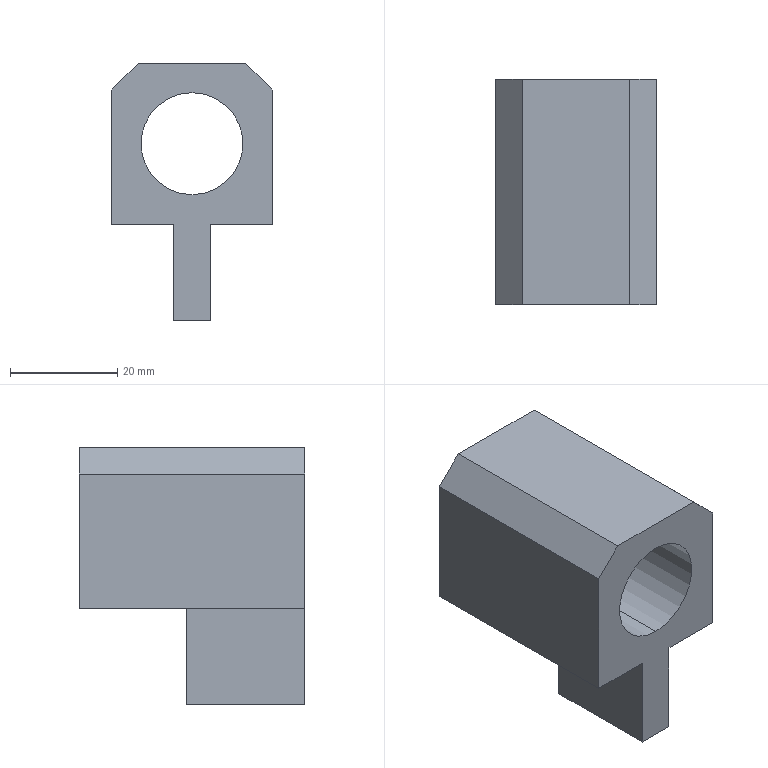Component | SolidWorks | STB-08-021-1 | 1 solid | 22 faces | box 30 x 42 x 48 mm | volume 27411 mm3 | plane 12 | cylinder 6 | cone 4 | commonest cylinder face diameters 3.3 x4 19 x2
build123d program:
from build123d import *

# Parameters (mm, degrees)
SKETCH1_W             = 30
SKETCH1_H             = 48
BOSS_EXTRUDE1_DEPTH   = 21
CUT_EXTRUDE1_REACH    = 52.646
SKETCH2_R             = 9.5
CUT_EXTRUDE2_REACH    = 52.646
SKETCH3_W             = 11.5
SKETCH3_H             = 18
M4_TAPPED_HOLE1_D     = 3.3
M4_TAPPED_HOLE1_DEPTH = 11.5
M4_TAPPED_HOLE1_TIP   = 0.9914
SKETCH7_W             = 7
SKETCH7_H             = 20
CUT_EXTRUDE4_DEPTH    = 18
CHAMFER1_SIZE         = 5


with BuildPart() as part:
    # Sketch1 → Boss-Extrude1 (new, symmetric)
    with BuildSketch(Plane(origin=(0, 0, 0), x_dir=(1, 0, 0), z_dir=(0, 1, 0))):
        Rectangle(SKETCH1_W, SKETCH1_H)
    extrude(amount=BOSS_EXTRUDE1_DEPTH, both=True)

    # Sketch2 → Cut-Extrude1 (cut, up to next)
    with BuildSketch(Plane(origin=(0, 21, 0), x_dir=(1, 0, 0), z_dir=(0, 1, 0)), mode=Mode.PRIVATE) as cut_extrude1_sk1:
        with Locations(Location((0, -9, 0), (0, 0, 270))):
            Circle(SKETCH2_R)
    cut_extrude1_tool1 = extrude(cut_extrude1_sk1.sketch, amount=-CUT_EXTRUDE1_REACH, mode=Mode.PRIVATE) & part.part
    add(cut_extrude1_tool1.solids().sort_by_distance((0, 21, 9))[0], mode=Mode.SUBTRACT)

    # Sketch3 → Cut-Extrude2 (cut, up to next)
    with BuildSketch(Plane(origin=(0, 21, 0), x_dir=(1, 0, 0), z_dir=(0, 1, 0)), mode=Mode.PRIVATE) as cut_extrude2_sk1:
        with Locations((-9.25, 15)):
            Rectangle(SKETCH3_W, SKETCH3_H)
    cut_extrude2_tool1 = extrude(cut_extrude2_sk1.sketch, amount=-CUT_EXTRUDE2_REACH, mode=Mode.PRIVATE) & part.part
    # Sketch3 → Cut-Extrude2 (cut, up to next)
    with BuildSketch(Plane(origin=(0, 21, 0), x_dir=(1, 0, 0), z_dir=(0, 1, 0)), mode=Mode.PRIVATE) as cut_extrude2_sk2:
        with Locations((9.25, 15)):
            Rectangle(SKETCH3_W, SKETCH3_H)
    cut_extrude2_tool2 = extrude(cut_extrude2_sk2.sketch, amount=-CUT_EXTRUDE2_REACH, mode=Mode.PRIVATE) & part.part
    add(cut_extrude2_tool1.solids().sort_by_distance((-9.25, 21, -15))[0], mode=Mode.SUBTRACT)
    add(cut_extrude2_tool2.solids().sort_by_distance((9.25, 21, -15))[0], mode=Mode.SUBTRACT)

    # M4 Tapped Hole1
    with Locations(Plane(origin=(0, 0, -24), x_dir=(-1, 0, 0), z_dir=(0, 0, -1))):
        with Locations((0, -15), (0, -5)):
            Hole(M4_TAPPED_HOLE1_D / 2, depth=M4_TAPPED_HOLE1_DEPTH)
            with Locations((0, 0, -(M4_TAPPED_HOLE1_DEPTH + M4_TAPPED_HOLE1_TIP / 2))):  # 118° drill point
                Cone(0, M4_TAPPED_HOLE1_D / 2, M4_TAPPED_HOLE1_TIP, mode=Mode.SUBTRACT)

    # Sketch7 → Cut-Extrude4 (cut)
    with BuildSketch(Plane(origin=(0, 0, -24), x_dir=(-1, 0, 0), z_dir=(0, 0, -1))):
        with Locations((0, 11)):
            Rectangle(SKETCH7_W, SKETCH7_H)
    extrude(amount=-CUT_EXTRUDE4_DEPTH, mode=Mode.SUBTRACT)

    # Chamfer1
    chamfer1_edges = [part.edges().sort_by_distance(p)[0] for p in [
        (15, 0, 24),
        (-15, 0, 24),
    ]]
    chamfer(chamfer1_edges, length=CHAMFER1_SIZE)


solid = part.part

# Placed as in the assembly
solid = solid.moved(Location((-149.904, 281.499, -21), (0, 0, 0)))
STEP:
#1=COLOUR_RGB('',0.7922,0.8196,0.9333);
#2=FILL_AREA_STYLE_COLOUR('',#1);
#3=FILL_AREA_STYLE('',(#2));
#4=SURFACE_STYLE_FILL_AREA(#3);
#5=SURFACE_SIDE_STYLE('',(#4));
#6=SURFACE_STYLE_USAGE(.BOTH.,#5);
#7=PRESENTATION_STYLE_ASSIGNMENT((#6));
#8=CARTESIAN_POINT('',(-5.837,10.492,-1.319));
#9=VERTEX_POINT('',#8);
#10=CARTESIAN_POINT('',(-5.967,10.492,-1.319));
#11=VERTEX_POINT('',#10);
#12=CARTESIAN_POINT('',(-5.902,10.492,-1.319));
#13=DIRECTION('',(0.,0.,-1.));
#14=DIRECTION('',(-1.,0.,0.));
#15=AXIS2_PLACEMENT_3D('',#12,#13,#14);
#16=CIRCLE('',#15,0.06496);
#17=EDGE_CURVE('',#9,#11,#16,.T.);
#18=ORIENTED_EDGE('',*,*,#17,.F.);
#19=CARTESIAN_POINT('',(-5.837,10.492,-1.772));
#20=VERTEX_POINT('',#19);
#21=CARTESIAN_POINT('',(-5.837,10.492,-1.772));
#22=DIRECTION('',(0.,0.,-1.));
#23=VECTOR('',#22,39.37);
#24=LINE('',#21,#23);
#25=EDGE_CURVE('',#9,#20,#24,.T.);
#26=ORIENTED_EDGE('',*,*,#25,.T.);
#27=CARTESIAN_POINT('',(-5.967,10.492,-1.772));
#28=VERTEX_POINT('',#27);
#29=CARTESIAN_POINT('',(-5.902,10.492,-1.772));
#30=DIRECTION('',(0.,0.,-1.));
#31=DIRECTION('',(-1.,0.,0.));
#32=AXIS2_PLACEMENT_3D('',#29,#30,#31);
#33=CIRCLE('',#32,0.06496);
#34=EDGE_CURVE('',#20,#28,#33,.T.);
#35=ORIENTED_EDGE('',*,*,#34,.T.);
#36=CARTESIAN_POINT('',(-5.967,10.492,-1.772));
#37=DIRECTION('',(0.,0.,-1.));
#38=VECTOR('',#37,39.37);
#39=LINE('',#36,#38);
#40=EDGE_CURVE('',#11,#28,#39,.T.);
#41=ORIENTED_EDGE('',*,*,#40,.F.);
#42=EDGE_LOOP('',(#18,#26,#35,#41));
#43=FACE_OUTER_BOUND('',#42,.T.);
#44=CARTESIAN_POINT('',(-5.902,10.492,-1.772));
#45=DIRECTION('',(0.,0.,-1.));
#46=DIRECTION('',(-1.,0.,0.));
#47=AXIS2_PLACEMENT_3D('',#44,#45,#46);
#48=CYLINDRICAL_SURFACE('',#47,0.06496);
#49=ADVANCED_FACE('',(#43),#48,.F.);
#50=CARTESIAN_POINT('',(-5.902,10.492,-1.28));
#51=VERTEX_POINT('',#50);
#52=CARTESIAN_POINT('',(-5.967,10.492,-1.319));
#53=DIRECTION('',(-0.8572,0.,-0.515));
#54=VECTOR('',#53,39.37);
#55=LINE('',#52,#54);
#56=EDGE_CURVE('',#51,#11,#55,.T.);
#57=ORIENTED_EDGE('',*,*,#56,.F.);
#58=CARTESIAN_POINT('',(-5.837,10.492,-1.319));
#59=DIRECTION('',(0.8572,0.,-0.515));
#60=VECTOR('',#59,39.37);
#61=LINE('',#58,#60);
#62=EDGE_CURVE('',#51,#9,#61,.T.);
#63=ORIENTED_EDGE('',*,*,#62,.T.);
#64=ORIENTED_EDGE('',*,*,#17,.T.);
#65=EDGE_LOOP('',(#57,#63,#64));
#66=FACE_OUTER_BOUND('',#65,.T.);
#67=CARTESIAN_POINT('',(-5.902,10.492,-1.319));
#68=DIRECTION('',(0.,0.,-1.));
#69=DIRECTION('',(-1.,0.,0.));
#70=AXIS2_PLACEMENT_3D('',#67,#68,#69);
#71=CONICAL_SURFACE('',#70,0.06496,1.03);
#72=ADVANCED_FACE('',(#66),#71,.F.);
#73=CARTESIAN_POINT('',(-5.837,10.886,-1.319));
#74=VERTEX_POINT('',#73);
#75=CARTESIAN_POINT('',(-5.967,10.886,-1.319));
#76=VERTEX_POINT('',#75);
#77=CARTESIAN_POINT('',(-5.902,10.886,-1.319));
#78=DIRECTION('',(0.,0.,-1.));
#79=DIRECTION('',(-1.,0.,0.));
#80=AXIS2_PLACEMENT_3D('',#77,#78,#79);
#81=CIRCLE('',#80,0.06496);
#82=EDGE_CURVE('',#74,#76,#81,.T.);
#83=ORIENTED_EDGE('',*,*,#82,.F.);
#84=CARTESIAN_POINT('',(-5.837,10.886,-1.772));
#85=VERTEX_POINT('',#84);
#86=CARTESIAN_POINT('',(-5.837,10.886,-1.772));
#87=DIRECTION('',(0.,0.,-1.));
#88=VECTOR('',#87,39.37);
#89=LINE('',#86,#88);
#90=EDGE_CURVE('',#74,#85,#89,.T.);
#91=ORIENTED_EDGE('',*,*,#90,.T.);
#92=CARTESIAN_POINT('',(-5.967,10.886,-1.772));
#93=VERTEX_POINT('',#92);
#94=CARTESIAN_POINT('',(-5.902,10.886,-1.772));
#95=DIRECTION('',(0.,0.,-1.));
#96=DIRECTION('',(-1.,0.,0.));
#97=AXIS2_PLACEMENT_3D('',#94,#95,#96);
#98=CIRCLE('',#97,0.06496);
#99=EDGE_CURVE('',#85,#93,#98,.T.);
#100=ORIENTED_EDGE('',*,*,#99,.T.);
#101=CARTESIAN_POINT('',(-5.967,10.886,-1.772));
#102=DIRECTION('',(0.,0.,-1.));
#103=VECTOR('',#102,39.37);
#104=LINE('',#101,#103);
#105=EDGE_CURVE('',#76,#93,#104,.T.);
#106=ORIENTED_EDGE('',*,*,#105,.F.);
#107=EDGE_LOOP('',(#83,#91,#100,#106));
#108=FACE_OUTER_BOUND('',#107,.T.);
#109=CARTESIAN_POINT('',(-5.902,10.886,-1.772));
#110=DIRECTION('',(0.,0.,-1.));
#111=DIRECTION('',(-1.,0.,0.));
#112=AXIS2_PLACEMENT_3D('',#109,#110,#111);
#113=CYLINDRICAL_SURFACE('',#112,0.06496);
#114=ADVANCED_FACE('',(#108),#113,.F.);
#115=CARTESIAN_POINT('',(-5.902,10.886,-1.28));
#116=VERTEX_POINT('',#115);
#117=CARTESIAN_POINT('',(-5.967,10.886,-1.319));
#118=DIRECTION('',(-0.8572,0.,-0.515));
#119=VECTOR('',#118,39.37);
#120=LINE('',#117,#119);
#121=EDGE_CURVE('',#116,#76,#120,.T.);
#122=ORIENTED_EDGE('',*,*,#121,.F.);
#123=CARTESIAN_POINT('',(-5.837,10.886,-1.319));
#124=DIRECTION('',(0.8572,0.,-0.515));
#125=VECTOR('',#124,39.37);
#126=LINE('',#123,#125);
#127=EDGE_CURVE('',#116,#74,#126,.T.);
#128=ORIENTED_EDGE('',*,*,#127,.T.);
#129=ORIENTED_EDGE('',*,*,#82,.T.);
#130=EDGE_LOOP('',(#122,#128,#129));
#131=FACE_OUTER_BOUND('',#130,.T.);
#132=CARTESIAN_POINT('',(-5.902,10.886,-1.319));
#133=DIRECTION('',(0.,0.,-1.));
#134=DIRECTION('',(-1.,0.,0.));
#135=AXIS2_PLACEMENT_3D('',#132,#133,#134);
#136=CONICAL_SURFACE('',#135,0.06496,1.03);
#137=ADVANCED_FACE('',(#131),#136,.F.);
#138=CARTESIAN_POINT('',(-5.902,10.256,-0.09843));
#139=VERTEX_POINT('',#138);
#140=CARTESIAN_POINT('',(-5.902,10.256,-0.8465));
#141=VERTEX_POINT('',#140);
#142=CARTESIAN_POINT('',(-5.902,10.256,-0.4724));
#143=DIRECTION('',(0.,-1.,0.));
#144=DIRECTION('',(0.,0.,1.));
#145=AXIS2_PLACEMENT_3D('',#142,#143,#144);
#146=CIRCLE('',#145,0.374);
#147=EDGE_CURVE('',#139,#141,#146,.T.);
#148=ORIENTED_EDGE('',*,*,#147,.T.);
#149=CARTESIAN_POINT('',(-5.902,11.909,-0.8465));
#150=VERTEX_POINT('',#149);
#151=CARTESIAN_POINT('',(-5.902,10.256,-0.8465));
#152=DIRECTION('',(0.,1.,0.));
#153=VECTOR('',#152,39.37);
#154=LINE('',#151,#153);
#155=EDGE_CURVE('',#141,#150,#154,.T.);
#156=ORIENTED_EDGE('',*,*,#155,.T.);
#157=CARTESIAN_POINT('',(-5.902,11.909,-0.09843));
#158=VERTEX_POINT('',#157);
#159=CARTESIAN_POINT('',(-5.902,11.909,-0.4724));
#160=DIRECTION('',(0.,1.,0.));
#161=DIRECTION('',(0.,0.,1.));
#162=AXIS2_PLACEMENT_3D('',#159,#160,#161);
#163=CIRCLE('',#162,0.374);
#164=EDGE_CURVE('',#150,#158,#163,.T.);
#165=ORIENTED_EDGE('',*,*,#164,.T.);
#166=CARTESIAN_POINT('',(-5.902,10.256,-0.09843));
#167=DIRECTION('',(0.,1.,0.));
#168=VECTOR('',#167,39.37);
#169=LINE('',#166,#168);
#170=EDGE_CURVE('',#139,#158,#169,.T.);
#171=ORIENTED_EDGE('',*,*,#170,.F.);
#172=EDGE_LOOP('',(#148,#156,#165,#171));
#173=FACE_OUTER_BOUND('',#172,.T.);
#174=CARTESIAN_POINT('',(-5.902,10.256,-0.4724));
#175=DIRECTION('',(0.,1.,0.));
#176=DIRECTION('',(0.,0.,1.));
#177=AXIS2_PLACEMENT_3D('',#174,#175,#176);
#178=CYLINDRICAL_SURFACE('',#177,0.374);
#179=ADVANCED_FACE('',(#173),#178,.F.);
#180=CARTESIAN_POINT('',(-5.902,11.909,-0.4724));
#181=DIRECTION('',(0.,1.,0.));
#182=DIRECTION('',(0.,0.,1.));
#183=AXIS2_PLACEMENT_3D('',#180,#181,#182);
#184=CIRCLE('',#183,0.374);
#185=EDGE_CURVE('',#158,#150,#184,.T.);
#186=ORIENTED_EDGE('',*,*,#185,.F.);
#187=ORIENTED_EDGE('',*,*,#164,.F.);
#188=EDGE_LOOP('',(#186,#187));
#189=FACE_BOUND('',#188,.T.);
#190=CARTESIAN_POINT('',(-6.492,11.909,-1.063));
#191=VERTEX_POINT('',#190);
#192=CARTESIAN_POINT('',(-6.492,11.909,-0.07874));
#193=VERTEX_POINT('',#192);
#194=CARTESIAN_POINT('',(-6.492,11.909,-1.772));
#195=DIRECTION('',(0.,0.,1.));
#196=VECTOR('',#195,39.37);
#197=LINE('',#194,#196);
#198=EDGE_CURVE('',#191,#193,#197,.T.);
#199=ORIENTED_EDGE('',*,*,#198,.T.);
#200=CARTESIAN_POINT('',(-6.295,11.909,0.1181));
#201=VERTEX_POINT('',#200);
#202=CARTESIAN_POINT('',(-6.394,11.909,0.01969));
#203=DIRECTION('',(0.7071,0.,0.7071));
#204=VECTOR('',#203,39.37);
#205=LINE('',#202,#204);
#206=EDGE_CURVE('',#193,#201,#205,.T.);
#207=ORIENTED_EDGE('',*,*,#206,.T.);
#208=CARTESIAN_POINT('',(-5.508,11.909,0.1181));
#209=VERTEX_POINT('',#208);
#210=CARTESIAN_POINT('',(-6.492,11.909,0.1181));
#211=DIRECTION('',(1.,0.,0.));
#212=VECTOR('',#211,39.37);
#213=LINE('',#210,#212);
#214=EDGE_CURVE('',#201,#209,#213,.T.);
#215=ORIENTED_EDGE('',*,*,#214,.T.);
#216=CARTESIAN_POINT('',(-5.311,11.909,-0.07874));
#217=VERTEX_POINT('',#216);
#218=CARTESIAN_POINT('',(-6.,11.909,0.6102));
#219=DIRECTION('',(0.7071,0.,-0.7071));
#220=VECTOR('',#219,39.37);
#221=LINE('',#218,#220);
#222=EDGE_CURVE('',#209,#217,#221,.T.);
#223=ORIENTED_EDGE('',*,*,#222,.T.);
#224=CARTESIAN_POINT('',(-5.311,11.909,-1.063));
#225=VERTEX_POINT('',#224);
#226=CARTESIAN_POINT('',(-5.311,11.909,-1.772));
#227=DIRECTION('',(0.,0.,-1.));
#228=VECTOR('',#227,39.37);
#229=LINE('',#226,#228);
#230=EDGE_CURVE('',#217,#225,#229,.T.);
#231=ORIENTED_EDGE('',*,*,#230,.T.);
#232=CARTESIAN_POINT('',(-6.492,11.909,-1.063));
#233=DIRECTION('',(1.,0.,0.));
#234=VECTOR('',#233,39.37);
#235=LINE('',#232,#234);
#236=EDGE_CURVE('',#191,#225,#235,.T.);
#237=ORIENTED_EDGE('',*,*,#236,.F.);
#238=EDGE_LOOP('',(#199,#207,#215,#223,#231,#237));
#239=FACE_OUTER_BOUND('',#238,.T.);
#240=CARTESIAN_POINT('',(-6.492,11.909,0.1181));
#241=DIRECTION('',(0.,1.,0.));
#242=DIRECTION('',(0.,0.,1.));
#243=AXIS2_PLACEMENT_3D('',#240,#241,#242);
#244=PLANE('',#243);
#245=ADVANCED_FACE('',(#189,#239),#244,.T.);
#246=CARTESIAN_POINT('',(-6.492,10.256,-1.063));
#247=VERTEX_POINT('',#246);
#248=CARTESIAN_POINT('',(-6.492,10.256,-0.07874));
#249=VERTEX_POINT('',#248);
#250=CARTESIAN_POINT('',(-6.492,10.256,-1.772));
#251=DIRECTION('',(0.,0.,1.));
#252=VECTOR('',#251,39.37);
#253=LINE('',#250,#252);
#254=EDGE_CURVE('',#247,#249,#253,.T.);
#255=ORIENTED_EDGE('',*,*,#254,.T.);
#256=CARTESIAN_POINT('',(-6.492,11.909,-0.07874));
#257=DIRECTION('',(0.,1.,0.));
#258=VECTOR('',#257,39.37);
#259=LINE('',#256,#258);
#260=EDGE_CURVE('',#249,#193,#259,.T.);
#261=ORIENTED_EDGE('',*,*,#260,.T.);
#262=ORIENTED_EDGE('',*,*,#198,.F.);
#263=CARTESIAN_POINT('',(-6.492,10.256,-1.063));
#264=DIRECTION('',(0.,1.,0.));
#265=VECTOR('',#264,39.37);
#266=LINE('',#263,#265);
#267=EDGE_CURVE('',#247,#191,#266,.T.);
#268=ORIENTED_EDGE('',*,*,#267,.F.);
#269=EDGE_LOOP('',(#255,#261,#262,#268));
#270=FACE_OUTER_BOUND('',#269,.T.);
#271=CARTESIAN_POINT('',(-6.492,11.909,-1.772));
#272=DIRECTION('',(1.,0.,0.));
#273=DIRECTION('',(0.,0.,-1.));
#274=AXIS2_PLACEMENT_3D('',#271,#272,#273);
#275=PLANE('',#274);
#276=ADVANCED_FACE('',(#270),#275,.F.);
#277=ORIENTED_EDGE('',*,*,#214,.F.);
#278=CARTESIAN_POINT('',(-6.295,10.256,0.1181));
#279=VERTEX_POINT('',#278);
#280=CARTESIAN_POINT('',(-6.295,11.909,0.1181));
#281=DIRECTION('',(0.,-1.,0.));
#282=VECTOR('',#281,39.37);
#283=LINE('',#280,#282);
#284=EDGE_CURVE('',#201,#279,#283,.T.);
#285=ORIENTED_EDGE('',*,*,#284,.T.);
#286=CARTESIAN_POINT('',(-5.508,10.256,0.1181));
#287=VERTEX_POINT('',#286);
#288=CARTESIAN_POINT('',(-6.492,10.256,0.1181));
#289=DIRECTION('',(1.,0.,0.));
#290=VECTOR('',#289,39.37);
#291=LINE('',#288,#290);
#292=EDGE_CURVE('',#279,#287,#291,.T.);
#293=ORIENTED_EDGE('',*,*,#292,.T.);
#294=CARTESIAN_POINT('',(-5.508,11.909,0.1181));
#295=DIRECTION('',(0.,1.,0.));
#296=VECTOR('',#295,39.37);
#297=LINE('',#294,#296);
#298=EDGE_CURVE('',#287,#209,#297,.T.);
#299=ORIENTED_EDGE('',*,*,#298,.T.);
#300=EDGE_LOOP('',(#277,#285,#293,#299));
#301=FACE_OUTER_BOUND('',#300,.T.);
#302=CARTESIAN_POINT('',(-6.492,11.909,0.1181));
#303=DIRECTION('',(0.,0.,-1.));
#304=DIRECTION('',(-1.,0.,0.));
#305=AXIS2_PLACEMENT_3D('',#302,#303,#304);
#306=PLANE('',#305);
#307=ADVANCED_FACE('',(#301),#306,.F.);
#308=ORIENTED_EDGE('',*,*,#230,.F.);
#309=CARTESIAN_POINT('',(-5.311,10.256,-0.07874));
#310=VERTEX_POINT('',#309);
#311=CARTESIAN_POINT('',(-5.311,11.909,-0.07874));
#312=DIRECTION('',(0.,-1.,0.));
#313=VECTOR('',#312,39.37);
#314=LINE('',#311,#313);
#315=EDGE_CURVE('',#217,#310,#314,.T.);
#316=ORIENTED_EDGE('',*,*,#315,.T.);
#317=CARTESIAN_POINT('',(-5.311,10.256,-1.063));
#318=VERTEX_POINT('',#317);
#319=CARTESIAN_POINT('',(-5.311,10.256,-1.772));
#320=DIRECTION('',(0.,0.,-1.));
#321=VECTOR('',#320,39.37);
#322=LINE('',#319,#321);
#323=EDGE_CURVE('',#310,#318,#322,.T.);
#324=ORIENTED_EDGE('',*,*,#323,.T.);
#325=CARTESIAN_POINT('',(-5.311,10.256,-1.063));
#326=DIRECTION('',(0.,1.,0.));
#327=VECTOR('',#326,39.37);
#328=LINE('',#325,#327);
#329=EDGE_CURVE('',#318,#225,#328,.T.);
#330=ORIENTED_EDGE('',*,*,#329,.T.);
#331=EDGE_LOOP('',(#308,#316,#324,#330));
#332=FACE_OUTER_BOUND('',#331,.T.);
#333=CARTESIAN_POINT('',(-5.311,11.909,-1.772));
#334=DIRECTION('',(-1.,0.,0.));
#335=DIRECTION('',(0.,0.,1.));
#336=AXIS2_PLACEMENT_3D('',#333,#334,#335);
#337=PLANE('',#336);
#338=ADVANCED_FACE('',(#332),#337,.F.);
#339=CARTESIAN_POINT('',(-5.902,10.492,-1.772));
#340=DIRECTION('',(0.,0.,-1.));
#341=DIRECTION('',(-1.,0.,0.));
#342=AXIS2_PLACEMENT_3D('',#339,#340,#341);
#343=CIRCLE('',#342,0.06496);
#344=EDGE_CURVE('',#28,#20,#343,.T.);
#345=ORIENTED_EDGE('',*,*,#344,.F.);
#346=ORIENTED_EDGE('',*,*,#34,.F.);
#347=EDGE_LOOP('',(#345,#346));
#348=FACE_BOUND('',#347,.T.);
#349=CARTESIAN_POINT('',(-5.902,10.886,-1.772));
#350=DIRECTION('',(0.,0.,-1.));
#351=DIRECTION('',(-1.,0.,0.));
#352=AXIS2_PLACEMENT_3D('',#349,#350,#351);
#353=CIRCLE('',#352,0.06496);
#354=EDGE_CURVE('',#93,#85,#353,.T.);
#355=ORIENTED_EDGE('',*,*,#354,.F.);
#356=ORIENTED_EDGE('',*,*,#99,.F.);
#357=EDGE_LOOP('',(#355,#356));
#358=FACE_BOUND('',#357,.T.);
#359=CARTESIAN_POINT('',(-6.04,10.256,-1.772));
#360=VERTEX_POINT('',#359);
#361=CARTESIAN_POINT('',(-6.04,11.122,-1.772));
#362=VERTEX_POINT('',#361);
#363=CARTESIAN_POINT('',(-6.04,10.256,-1.772));
#364=DIRECTION('',(0.,1.,0.));
#365=VECTOR('',#364,39.37);
#366=LINE('',#363,#365);
#367=EDGE_CURVE('',#360,#362,#366,.T.);
#368=ORIENTED_EDGE('',*,*,#367,.T.);
#369=CARTESIAN_POINT('',(-5.764,11.122,-1.772));
#370=VERTEX_POINT('',#369);
#371=CARTESIAN_POINT('',(-5.764,11.122,-1.772));
#372=DIRECTION('',(-1.,0.,0.));
#373=VECTOR('',#372,39.37);
#374=LINE('',#371,#373);
#375=EDGE_CURVE('',#370,#362,#374,.T.);
#376=ORIENTED_EDGE('',*,*,#375,.F.);
#377=CARTESIAN_POINT('',(-5.764,10.256,-1.772));
#378=VERTEX_POINT('',#377);
#379=CARTESIAN_POINT('',(-5.764,10.256,-1.772));
#380=DIRECTION('',(0.,1.,0.));
#381=VECTOR('',#380,39.37);
#382=LINE('',#379,#381);
#383=EDGE_CURVE('',#378,#370,#382,.T.);
#384=ORIENTED_EDGE('',*,*,#383,.F.);
#385=CARTESIAN_POINT('',(-6.492,10.256,-1.772));
#386=DIRECTION('',(-1.,0.,0.));
#387=VECTOR('',#386,39.37);
#388=LINE('',#385,#387);
#389=EDGE_CURVE('',#378,#360,#388,.T.);
#390=ORIENTED_EDGE('',*,*,#389,.T.);
#391=EDGE_LOOP('',(#368,#376,#384,#390));
#392=FACE_OUTER_BOUND('',#391,.T.);
#393=CARTESIAN_POINT('',(-6.492,11.909,-1.772));
#394=DIRECTION('',(0.,0.,1.));
#395=DIRECTION('',(1.,0.,0.));
#396=AXIS2_PLACEMENT_3D('',#393,#394,#395);
#397=PLANE('',#396);
#398=ADVANCED_FACE('',(#348,#358,#392),#397,.F.);
#399=ORIENTED_EDGE('',*,*,#147,.F.);
#400=CARTESIAN_POINT('',(-5.902,10.256,-0.4724));
#401=DIRECTION('',(0.,-1.,0.));
#402=DIRECTION('',(0.,0.,1.));
#403=AXIS2_PLACEMENT_3D('',#400,#401,#402);
#404=CIRCLE('',#403,0.374);
#405=EDGE_CURVE('',#141,#139,#404,.T.);
#406=ORIENTED_EDGE('',*,*,#405,.F.);
#407=EDGE_LOOP('',(#399,#406));
#408=FACE_BOUND('',#407,.T.);
#409=ORIENTED_EDGE('',*,*,#292,.F.);
#410=CARTESIAN_POINT('',(-6.295,10.256,0.1181));
#411=DIRECTION('',(-0.7071,0.,-0.7071));
#412=VECTOR('',#411,39.37);
#413=LINE('',#410,#412);
#414=EDGE_CURVE('',#279,#249,#413,.T.);
#415=ORIENTED_EDGE('',*,*,#414,.T.);
#416=ORIENTED_EDGE('',*,*,#254,.F.);
#417=CARTESIAN_POINT('',(-6.04,10.256,-1.063));
#418=VERTEX_POINT('',#417);
#419=CARTESIAN_POINT('',(-6.492,10.256,-1.063));
#420=DIRECTION('',(-1.,0.,-0.));
#421=VECTOR('',#420,39.37);
#422=LINE('',#419,#421);
#423=EDGE_CURVE('',#418,#247,#422,.T.);
#424=ORIENTED_EDGE('',*,*,#423,.F.);
#425=CARTESIAN_POINT('',(-6.04,10.256,-1.772));
#426=DIRECTION('',(-0.,0.,1.));
#427=VECTOR('',#426,39.37);
#428=LINE('',#425,#427);
#429=EDGE_CURVE('',#360,#418,#428,.T.);
#430=ORIENTED_EDGE('',*,*,#429,.F.);
#431=ORIENTED_EDGE('',*,*,#389,.F.);
#432=CARTESIAN_POINT('',(-5.764,10.256,-1.063));
#433=VERTEX_POINT('',#432);
#434=CARTESIAN_POINT('',(-5.764,10.256,-1.772));
#435=DIRECTION('',(-0.,0.,-1.));
#436=VECTOR('',#435,39.37);
#437=LINE('',#434,#436);
#438=EDGE_CURVE('',#433,#378,#437,.T.);
#439=ORIENTED_EDGE('',*,*,#438,.F.);
#440=CARTESIAN_POINT('',(-5.311,10.256,-1.063));
#441=DIRECTION('',(-1.,0.,0.));
#442=VECTOR('',#441,39.37);
#443=LINE('',#440,#442);
#444=EDGE_CURVE('',#318,#433,#443,.T.);
#445=ORIENTED_EDGE('',*,*,#444,.F.);
#446=ORIENTED_EDGE('',*,*,#323,.F.);
#447=CARTESIAN_POINT('',(-5.311,10.256,-0.07874));
#448=DIRECTION('',(-0.7071,0.,0.7071));
#449=VECTOR('',#448,39.37);
#450=LINE('',#447,#449);
#451=EDGE_CURVE('',#310,#287,#450,.T.);
#452=ORIENTED_EDGE('',*,*,#451,.T.);
#453=EDGE_LOOP('',(#409,#415,#416,#424,#430,#431,#439,#445,#446,#452));
#454=FACE_OUTER_BOUND('',#453,.T.);
#455=CARTESIAN_POINT('',(-6.492,10.256,0.1181));
#456=DIRECTION('',(0.,1.,0.));
#457=DIRECTION('',(0.,0.,1.));
#458=AXIS2_PLACEMENT_3D('',#455,#456,#457);
#459=PLANE('',#458);
#460=ADVANCED_FACE('',(#408,#454),#459,.F.);
#461=ORIENTED_EDGE('',*,*,#155,.F.);
#462=ORIENTED_EDGE('',*,*,#405,.T.);
#463=ORIENTED_EDGE('',*,*,#170,.T.);
#464=ORIENTED_EDGE('',*,*,#185,.T.);
#465=EDGE_LOOP('',(#461,#462,#463,#464));
#466=FACE_OUTER_BOUND('',#465,.T.);
#467=CARTESIAN_POINT('',(-5.902,10.256,-0.4724));
#468=DIRECTION('',(0.,1.,0.));
#469=DIRECTION('',(0.,0.,1.));
#470=AXIS2_PLACEMENT_3D('',#467,#468,#469);
#471=CYLINDRICAL_SURFACE('',#470,0.374);
#472=ADVANCED_FACE('',(#466),#471,.F.);
#473=CARTESIAN_POINT('',(-6.04,11.122,-1.063));
#474=VERTEX_POINT('',#473);
#475=CARTESIAN_POINT('',(-6.04,10.256,-1.063));
#476=DIRECTION('',(0.,1.,0.));
#477=VECTOR('',#476,39.37);
#478=LINE('',#475,#477);
#479=EDGE_CURVE('',#418,#474,#478,.T.);
#480=ORIENTED_EDGE('',*,*,#479,.T.);
#481=CARTESIAN_POINT('',(-6.04,11.122,-1.063));
#482=DIRECTION('',(0.,0.,-1.));
#483=VECTOR('',#482,39.37);
#484=LINE('',#481,#483);
#485=EDGE_CURVE('',#474,#362,#484,.T.);
#486=ORIENTED_EDGE('',*,*,#485,.T.);
#487=ORIENTED_EDGE('',*,*,#367,.F.);
#488=ORIENTED_EDGE('',*,*,#429,.T.);
#489=EDGE_LOOP('',(#480,#486,#487,#488));
#490=FACE_OUTER_BOUND('',#489,.T.);
#491=CARTESIAN_POINT('',(-6.04,10.256,-1.772));
#492=DIRECTION('',(1.,0.,0.));
#493=DIRECTION('',(0.,0.,-1.));
#494=AXIS2_PLACEMENT_3D('',#491,#492,#493);
#495=PLANE('',#494);
#496=ADVANCED_FACE('',(#490),#495,.F.);
#497=ORIENTED_EDGE('',*,*,#423,.T.);
#498=ORIENTED_EDGE('',*,*,#267,.T.);
#499=ORIENTED_EDGE('',*,*,#236,.T.);
#500=ORIENTED_EDGE('',*,*,#329,.F.);
#501=ORIENTED_EDGE('',*,*,#444,.T.);
#502=CARTESIAN_POINT('',(-5.764,11.122,-1.063));
#503=VERTEX_POINT('',#502);
#504=CARTESIAN_POINT('',(-5.764,10.256,-1.063));
#505=DIRECTION('',(0.,1.,0.));
#506=VECTOR('',#505,39.37);
#507=LINE('',#504,#506);
#508=EDGE_CURVE('',#433,#503,#507,.T.);
#509=ORIENTED_EDGE('',*,*,#508,.T.);
#510=CARTESIAN_POINT('',(-5.764,11.122,-1.063));
#511=DIRECTION('',(-1.,0.,0.));
#512=VECTOR('',#511,39.37);
#513=LINE('',#510,#512);
#514=EDGE_CURVE('',#503,#474,#513,.T.);
#515=ORIENTED_EDGE('',*,*,#514,.T.);
#516=ORIENTED_EDGE('',*,*,#479,.F.);
#517=EDGE_LOOP('',(#497,#498,#499,#500,#501,#509,#515,#516));
#518=FACE_OUTER_BOUND('',#517,.T.);
#519=CARTESIAN_POINT('',(-6.492,10.256,-1.063));
#520=DIRECTION('',(-0.,0.,1.));
#521=DIRECTION('',(1.,0.,0.));
#522=AXIS2_PLACEMENT_3D('',#519,#520,#521);
#523=PLANE('',#522);
#524=ADVANCED_FACE('',(#518),#523,.F.);
#525=ORIENTED_EDGE('',*,*,#383,.T.);
#526=CARTESIAN_POINT('',(-5.764,11.122,-1.063));
#527=DIRECTION('',(0.,0.,-1.));
#528=VECTOR('',#527,39.37);
#529=LINE('',#526,#528);
#530=EDGE_CURVE('',#503,#370,#529,.T.);
#531=ORIENTED_EDGE('',*,*,#530,.F.);
#532=ORIENTED_EDGE('',*,*,#508,.F.);
#533=ORIENTED_EDGE('',*,*,#438,.T.);
#534=EDGE_LOOP('',(#525,#531,#532,#533));
#535=FACE_OUTER_BOUND('',#534,.T.);
#536=CARTESIAN_POINT('',(-5.764,10.256,-1.772));
#537=DIRECTION('',(-1.,0.,0.));
#538=DIRECTION('',(0.,0.,1.));
#539=AXIS2_PLACEMENT_3D('',#536,#537,#538);
#540=PLANE('',#539);
#541=ADVANCED_FACE('',(#535),#540,.F.);
#542=ORIENTED_EDGE('',*,*,#127,.F.);
#543=ORIENTED_EDGE('',*,*,#121,.T.);
#544=CARTESIAN_POINT('',(-5.902,10.886,-1.319));
#545=DIRECTION('',(0.,0.,-1.));
#546=DIRECTION('',(-1.,0.,0.));
#547=AXIS2_PLACEMENT_3D('',#544,#545,#546);
#548=CIRCLE('',#547,0.06496);
#549=EDGE_CURVE('',#76,#74,#548,.T.);
#550=ORIENTED_EDGE('',*,*,#549,.T.);
#551=EDGE_LOOP('',(#542,#543,#550));
#552=FACE_OUTER_BOUND('',#551,.T.);
#553=CARTESIAN_POINT('',(-5.902,10.886,-1.319));
#554=DIRECTION('',(0.,0.,-1.));
#555=DIRECTION('',(-1.,0.,0.));
#556=AXIS2_PLACEMENT_3D('',#553,#554,#555);
#557=CONICAL_SURFACE('',#556,0.06496,1.03);
#558=ADVANCED_FACE('',(#552),#557,.F.);
#559=ORIENTED_EDGE('',*,*,#90,.F.);
#560=ORIENTED_EDGE('',*,*,#549,.F.);
#561=ORIENTED_EDGE('',*,*,#105,.T.);
#562=ORIENTED_EDGE('',*,*,#354,.T.);
#563=EDGE_LOOP('',(#559,#560,#561,#562));
#564=FACE_OUTER_BOUND('',#563,.T.);
#565=CARTESIAN_POINT('',(-5.902,10.886,-1.772));
#566=DIRECTION('',(0.,0.,-1.));
#567=DIRECTION('',(-1.,0.,0.));
#568=AXIS2_PLACEMENT_3D('',#565,#566,#567);
#569=CYLINDRICAL_SURFACE('',#568,0.06496);
#570=ADVANCED_FACE('',(#564),#569,.F.);
#571=ORIENTED_EDGE('',*,*,#62,.F.);
#572=ORIENTED_EDGE('',*,*,#56,.T.);
#573=CARTESIAN_POINT('',(-5.902,10.492,-1.319));
#574=DIRECTION('',(0.,0.,-1.));
#575=DIRECTION('',(-1.,0.,0.));
#576=AXIS2_PLACEMENT_3D('',#573,#574,#575);
#577=CIRCLE('',#576,0.06496);
#578=EDGE_CURVE('',#11,#9,#577,.T.);
#579=ORIENTED_EDGE('',*,*,#578,.T.);
#580=EDGE_LOOP('',(#571,#572,#579));
#581=FACE_OUTER_BOUND('',#580,.T.);
#582=CARTESIAN_POINT('',(-5.902,10.492,-1.319));
#583=DIRECTION('',(0.,0.,-1.));
#584=DIRECTION('',(-1.,0.,0.));
#585=AXIS2_PLACEMENT_3D('',#582,#583,#584);
#586=CONICAL_SURFACE('',#585,0.06496,1.03);
#587=ADVANCED_FACE('',(#581),#586,.F.);
#588=ORIENTED_EDGE('',*,*,#25,.F.);
#589=ORIENTED_EDGE('',*,*,#578,.F.);
#590=ORIENTED_EDGE('',*,*,#40,.T.);
#591=ORIENTED_EDGE('',*,*,#344,.T.);
#592=EDGE_LOOP('',(#588,#589,#590,#591));
#593=FACE_OUTER_BOUND('',#592,.T.);
#594=CARTESIAN_POINT('',(-5.902,10.492,-1.772));
#595=DIRECTION('',(0.,0.,-1.));
#596=DIRECTION('',(-1.,0.,0.));
#597=AXIS2_PLACEMENT_3D('',#594,#595,#596);
#598=CYLINDRICAL_SURFACE('',#597,0.06496);
#599=ADVANCED_FACE('',(#593),#598,.F.);
#600=ORIENTED_EDGE('',*,*,#375,.T.);
#601=ORIENTED_EDGE('',*,*,#485,.F.);
#602=ORIENTED_EDGE('',*,*,#514,.F.);
#603=ORIENTED_EDGE('',*,*,#530,.T.);
#604=EDGE_LOOP('',(#600,#601,#602,#603));
#605=FACE_OUTER_BOUND('',#604,.T.);
#606=CARTESIAN_POINT('',(-5.764,11.122,-1.063));
#607=DIRECTION('',(0.,-1.,0.));
#608=DIRECTION('',(0.,0.,-1.));
#609=AXIS2_PLACEMENT_3D('',#606,#607,#608);
#610=PLANE('',#609);
#611=ADVANCED_FACE('',(#605),#610,.F.);
#612=ORIENTED_EDGE('',*,*,#206,.F.);
#613=ORIENTED_EDGE('',*,*,#260,.F.);
#614=ORIENTED_EDGE('',*,*,#414,.F.);
#615=ORIENTED_EDGE('',*,*,#284,.F.);
#616=EDGE_LOOP('',(#612,#613,#614,#615));
#617=FACE_OUTER_BOUND('',#616,.T.);
#618=CARTESIAN_POINT('',(-6.295,11.909,0.1181));
#619=DIRECTION('',(0.7071,0.,-0.7071));
#620=DIRECTION('',(-0.7071,0.,-0.7071));
#621=AXIS2_PLACEMENT_3D('',#618,#619,#620);
#622=PLANE('',#621);
#623=ADVANCED_FACE('',(#617),#622,.F.);
#624=ORIENTED_EDGE('',*,*,#222,.F.);
#625=ORIENTED_EDGE('',*,*,#298,.F.);
#626=ORIENTED_EDGE('',*,*,#451,.F.);
#627=ORIENTED_EDGE('',*,*,#315,.F.);
#628=EDGE_LOOP('',(#624,#625,#626,#627));
#629=FACE_OUTER_BOUND('',#628,.T.);
#630=CARTESIAN_POINT('',(-5.311,11.909,-0.07874));
#631=DIRECTION('',(-0.7071,0.,-0.7071));
#632=DIRECTION('',(-0.7071,0.,0.7071));
#633=AXIS2_PLACEMENT_3D('',#630,#631,#632);
#634=PLANE('',#633);
#635=ADVANCED_FACE('',(#629),#634,.F.);
#636=CLOSED_SHELL('',(#49,#72,#114,#137,#179,#245,#276,#307,#338,#398,#460,#472,#496,#524,#541,#558,#570,#587,#599,#611,#623,#635));
#637=MANIFOLD_SOLID_BREP('',#636);
#638=STYLED_ITEM('',(#7),#637);
#639=PRESENTATION_LAYER_ASSIGNMENT('','',(#638));
#640=(LENGTH_UNIT()NAMED_UNIT(*)SI_UNIT($,.METRE.));
#641=LENGTH_MEASURE_WITH_UNIT(LENGTH_MEASURE(0.0254),#640);
#642=DIMENSIONAL_EXPONENTS(1.,0.,0.,0.,0.,0.,0.);
#643=(CONVERSION_BASED_UNIT('',#641)LENGTH_UNIT()NAMED_UNIT(#642));
#644=UNCERTAINTY_MEASURE_WITH_UNIT(LENGTH_MEASURE(0.00001),#643,'','');
#645=(NAMED_UNIT(*)PLANE_ANGLE_UNIT()SI_UNIT($,.RADIAN.));
#646=(NAMED_UNIT(*)SI_UNIT($,.STERADIAN.)SOLID_ANGLE_UNIT());
#647=(GEOMETRIC_REPRESENTATION_CONTEXT(3)GLOBAL_UNCERTAINTY_ASSIGNED_CONTEXT((#644))GLOBAL_UNIT_ASSIGNED_CONTEXT((#643,#645,#646))REPRESENTATION_CONTEXT('',''));
#648=MECHANICAL_DESIGN_GEOMETRIC_PRESENTATION_REPRESENTATION('',(#638),#647);
#649=CARTESIAN_POINT('',(0.,0.,0.));
#650=DIRECTION('',(0.,0.,1.));
#651=DIRECTION('',(1.,0.,0.));
#652=AXIS2_PLACEMENT_3D('',#649,#650,#651);
#653=(LENGTH_UNIT()NAMED_UNIT(*)SI_UNIT($,.METRE.));
#654=LENGTH_MEASURE_WITH_UNIT(LENGTH_MEASURE(0.0254),#653);
#655=DIMENSIONAL_EXPONENTS(1.,0.,0.,0.,0.,0.,0.);
#656=(CONVERSION_BASED_UNIT('',#654)LENGTH_UNIT()NAMED_UNIT(#655));
#657=UNCERTAINTY_MEASURE_WITH_UNIT(LENGTH_MEASURE(0.00001),#656,'','');
#658=(NAMED_UNIT(*)PLANE_ANGLE_UNIT()SI_UNIT($,.RADIAN.));
#659=(NAMED_UNIT(*)SI_UNIT($,.STERADIAN.)SOLID_ANGLE_UNIT());
#660=(GEOMETRIC_REPRESENTATION_CONTEXT(3)GLOBAL_UNCERTAINTY_ASSIGNED_CONTEXT((#657))GLOBAL_UNIT_ASSIGNED_CONTEXT((#656,#658,#659))REPRESENTATION_CONTEXT('',''));
#661=ADVANCED_BREP_SHAPE_REPRESENTATION('',(#637,#652),#660);